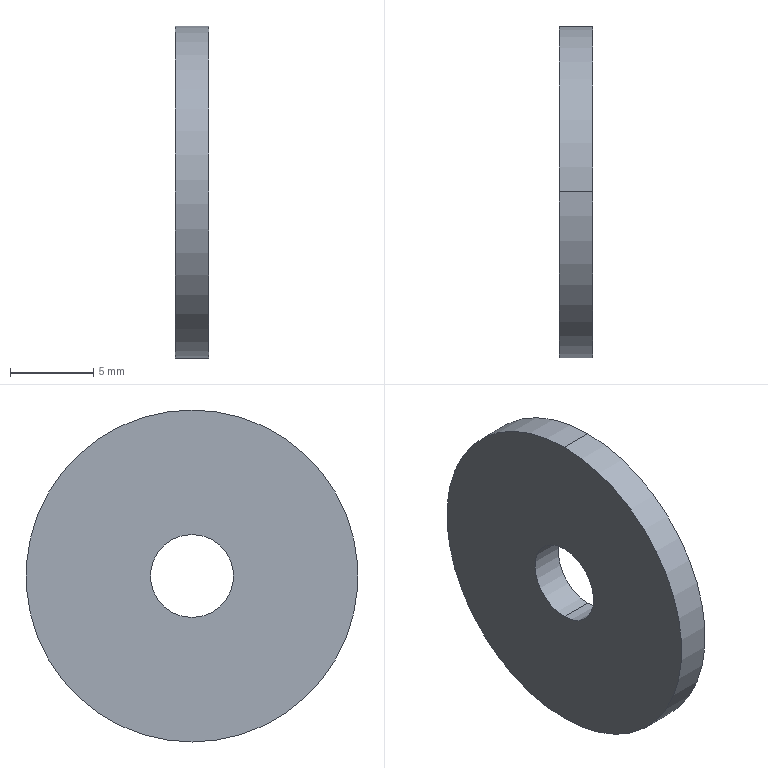Component | SolidWorks | Baffle2-1 | 1 solid | 6 faces | box 2 x 20 x 20 mm | volume 589 mm3 | cylinder 4 | plane 2 | commonest cylinder face diameters 5 x2 20 x2
STEP:
#1=COLOUR_RGB('',0.7922,0.8196,0.9333);
#2=FILL_AREA_STYLE_COLOUR('',#1);
#3=FILL_AREA_STYLE('',(#2));
#4=SURFACE_STYLE_FILL_AREA(#3);
#5=SURFACE_SIDE_STYLE('',(#4));
#6=SURFACE_STYLE_USAGE(.BOTH.,#5);
#7=PRESENTATION_STYLE_ASSIGNMENT((#6));
#8=CARTESIAN_POINT('',(-9.665,5.032,3.217));
#9=VERTEX_POINT('',#8);
#10=CARTESIAN_POINT('',(-9.665,5.032,3.02));
#11=VERTEX_POINT('',#10);
#12=CARTESIAN_POINT('',(-9.665,5.032,3.119));
#13=DIRECTION('',(1.,0.,0.));
#14=DIRECTION('',(0.,0.,-1.));
#15=AXIS2_PLACEMENT_3D('',#12,#13,#14);
#16=CIRCLE('',#15,0.09843);
#17=EDGE_CURVE('',#9,#11,#16,.T.);
#18=ORIENTED_EDGE('',*,*,#17,.F.);
#19=CARTESIAN_POINT('',(-9.587,5.032,3.217));
#20=VERTEX_POINT('',#19);
#21=CARTESIAN_POINT('',(-9.665,5.032,3.217));
#22=DIRECTION('',(1.,0.,0.));
#23=VECTOR('',#22,39.37);
#24=LINE('',#21,#23);
#25=EDGE_CURVE('',#9,#20,#24,.T.);
#26=ORIENTED_EDGE('',*,*,#25,.T.);
#27=CARTESIAN_POINT('',(-9.587,5.032,3.02));
#28=VERTEX_POINT('',#27);
#29=CARTESIAN_POINT('',(-9.587,5.032,3.119));
#30=DIRECTION('',(1.,0.,0.));
#31=DIRECTION('',(0.,0.,-1.));
#32=AXIS2_PLACEMENT_3D('',#29,#30,#31);
#33=CIRCLE('',#32,0.09843);
#34=EDGE_CURVE('',#20,#28,#33,.T.);
#35=ORIENTED_EDGE('',*,*,#34,.T.);
#36=CARTESIAN_POINT('',(-9.665,5.032,3.02));
#37=DIRECTION('',(1.,0.,0.));
#38=VECTOR('',#37,39.37);
#39=LINE('',#36,#38);
#40=EDGE_CURVE('',#11,#28,#39,.T.);
#41=ORIENTED_EDGE('',*,*,#40,.F.);
#42=EDGE_LOOP('',(#18,#26,#35,#41));
#43=FACE_OUTER_BOUND('',#42,.T.);
#44=CARTESIAN_POINT('',(-9.665,5.032,3.119));
#45=DIRECTION('',(1.,0.,0.));
#46=DIRECTION('',(0.,0.,-1.));
#47=AXIS2_PLACEMENT_3D('',#44,#45,#46);
#48=CYLINDRICAL_SURFACE('',#47,0.09843);
#49=ADVANCED_FACE('',(#43),#48,.F.);
#50=CARTESIAN_POINT('',(-9.665,5.032,2.725));
#51=VERTEX_POINT('',#50);
#52=CARTESIAN_POINT('',(-9.665,5.032,3.512));
#53=VERTEX_POINT('',#52);
#54=CARTESIAN_POINT('',(-9.665,5.032,3.119));
#55=DIRECTION('',(1.,0.,0.));
#56=DIRECTION('',(0.,0.,-1.));
#57=AXIS2_PLACEMENT_3D('',#54,#55,#56);
#58=CIRCLE('',#57,0.3937);
#59=EDGE_CURVE('',#51,#53,#58,.T.);
#60=ORIENTED_EDGE('',*,*,#59,.T.);
#61=CARTESIAN_POINT('',(-9.587,5.032,3.512));
#62=VERTEX_POINT('',#61);
#63=CARTESIAN_POINT('',(-9.665,5.032,3.512));
#64=DIRECTION('',(1.,0.,0.));
#65=VECTOR('',#64,39.37);
#66=LINE('',#63,#65);
#67=EDGE_CURVE('',#53,#62,#66,.T.);
#68=ORIENTED_EDGE('',*,*,#67,.T.);
#69=CARTESIAN_POINT('',(-9.587,5.032,2.725));
#70=VERTEX_POINT('',#69);
#71=CARTESIAN_POINT('',(-9.587,5.032,3.119));
#72=DIRECTION('',(1.,0.,0.));
#73=DIRECTION('',(0.,0.,-1.));
#74=AXIS2_PLACEMENT_3D('',#71,#72,#73);
#75=CIRCLE('',#74,0.3937);
#76=EDGE_CURVE('',#70,#62,#75,.T.);
#77=ORIENTED_EDGE('',*,*,#76,.F.);
#78=CARTESIAN_POINT('',(-9.665,5.032,2.725));
#79=DIRECTION('',(1.,0.,0.));
#80=VECTOR('',#79,39.37);
#81=LINE('',#78,#80);
#82=EDGE_CURVE('',#51,#70,#81,.T.);
#83=ORIENTED_EDGE('',*,*,#82,.F.);
#84=EDGE_LOOP('',(#60,#68,#77,#83));
#85=FACE_OUTER_BOUND('',#84,.T.);
#86=CARTESIAN_POINT('',(-9.665,5.032,3.119));
#87=DIRECTION('',(1.,0.,0.));
#88=DIRECTION('',(0.,0.,-1.));
#89=AXIS2_PLACEMENT_3D('',#86,#87,#88);
#90=CYLINDRICAL_SURFACE('',#89,0.3937);
#91=ADVANCED_FACE('',(#85),#90,.T.);
#92=ORIENTED_EDGE('',*,*,#67,.F.);
#93=CARTESIAN_POINT('',(-9.665,5.032,3.119));
#94=DIRECTION('',(1.,0.,0.));
#95=DIRECTION('',(0.,0.,-1.));
#96=AXIS2_PLACEMENT_3D('',#93,#94,#95);
#97=CIRCLE('',#96,0.3937);
#98=EDGE_CURVE('',#53,#51,#97,.T.);
#99=ORIENTED_EDGE('',*,*,#98,.T.);
#100=ORIENTED_EDGE('',*,*,#82,.T.);
#101=CARTESIAN_POINT('',(-9.587,5.032,3.119));
#102=DIRECTION('',(1.,0.,0.));
#103=DIRECTION('',(0.,0.,-1.));
#104=AXIS2_PLACEMENT_3D('',#101,#102,#103);
#105=CIRCLE('',#104,0.3937);
#106=EDGE_CURVE('',#62,#70,#105,.T.);
#107=ORIENTED_EDGE('',*,*,#106,.F.);
#108=EDGE_LOOP('',(#92,#99,#100,#107));
#109=FACE_OUTER_BOUND('',#108,.T.);
#110=CARTESIAN_POINT('',(-9.665,5.032,3.119));
#111=DIRECTION('',(1.,0.,0.));
#112=DIRECTION('',(0.,0.,-1.));
#113=AXIS2_PLACEMENT_3D('',#110,#111,#112);
#114=CYLINDRICAL_SURFACE('',#113,0.3937);
#115=ADVANCED_FACE('',(#109),#114,.T.);
#116=CARTESIAN_POINT('',(-9.665,5.032,3.119));
#117=DIRECTION('',(1.,0.,0.));
#118=DIRECTION('',(0.,0.,-1.));
#119=AXIS2_PLACEMENT_3D('',#116,#117,#118);
#120=CIRCLE('',#119,0.09843);
#121=EDGE_CURVE('',#11,#9,#120,.T.);
#122=ORIENTED_EDGE('',*,*,#121,.T.);
#123=ORIENTED_EDGE('',*,*,#17,.T.);
#124=EDGE_LOOP('',(#122,#123));
#125=FACE_BOUND('',#124,.T.);
#126=ORIENTED_EDGE('',*,*,#59,.F.);
#127=ORIENTED_EDGE('',*,*,#98,.F.);
#128=EDGE_LOOP('',(#126,#127));
#129=FACE_OUTER_BOUND('',#128,.T.);
#130=CARTESIAN_POINT('',(-9.665,5.032,3.119));
#131=DIRECTION('',(1.,0.,0.));
#132=DIRECTION('',(0.,0.,-1.));
#133=AXIS2_PLACEMENT_3D('',#130,#131,#132);
#134=PLANE('',#133);
#135=ADVANCED_FACE('',(#125,#129),#134,.F.);
#136=CARTESIAN_POINT('',(-9.587,5.032,3.119));
#137=DIRECTION('',(1.,0.,0.));
#138=DIRECTION('',(0.,0.,-1.));
#139=AXIS2_PLACEMENT_3D('',#136,#137,#138);
#140=CIRCLE('',#139,0.09843);
#141=EDGE_CURVE('',#28,#20,#140,.T.);
#142=ORIENTED_EDGE('',*,*,#141,.F.);
#143=ORIENTED_EDGE('',*,*,#34,.F.);
#144=EDGE_LOOP('',(#142,#143));
#145=FACE_BOUND('',#144,.T.);
#146=ORIENTED_EDGE('',*,*,#76,.T.);
#147=ORIENTED_EDGE('',*,*,#106,.T.);
#148=EDGE_LOOP('',(#146,#147));
#149=FACE_OUTER_BOUND('',#148,.T.);
#150=CARTESIAN_POINT('',(-9.587,5.032,3.119));
#151=DIRECTION('',(1.,0.,0.));
#152=DIRECTION('',(0.,0.,-1.));
#153=AXIS2_PLACEMENT_3D('',#150,#151,#152);
#154=PLANE('',#153);
#155=ADVANCED_FACE('',(#145,#149),#154,.T.);
#156=ORIENTED_EDGE('',*,*,#25,.F.);
#157=ORIENTED_EDGE('',*,*,#121,.F.);
#158=ORIENTED_EDGE('',*,*,#40,.T.);
#159=ORIENTED_EDGE('',*,*,#141,.T.);
#160=EDGE_LOOP('',(#156,#157,#158,#159));
#161=FACE_OUTER_BOUND('',#160,.T.);
#162=CARTESIAN_POINT('',(-9.665,5.032,3.119));
#163=DIRECTION('',(1.,0.,0.));
#164=DIRECTION('',(0.,0.,-1.));
#165=AXIS2_PLACEMENT_3D('',#162,#163,#164);
#166=CYLINDRICAL_SURFACE('',#165,0.09843);
#167=ADVANCED_FACE('',(#161),#166,.F.);
#168=CLOSED_SHELL('',(#49,#91,#115,#135,#155,#167));
#169=MANIFOLD_SOLID_BREP('',#168);
#170=STYLED_ITEM('',(#7),#169);
#171=(LENGTH_UNIT()NAMED_UNIT(*)SI_UNIT($,.METRE.));
#172=LENGTH_MEASURE_WITH_UNIT(LENGTH_MEASURE(0.0254),#171);
#173=DIMENSIONAL_EXPONENTS(1.,0.,0.,0.,0.,0.,0.);
#174=(CONVERSION_BASED_UNIT('',#172)LENGTH_UNIT()NAMED_UNIT(#173));
#175=UNCERTAINTY_MEASURE_WITH_UNIT(LENGTH_MEASURE(0.00001),#174,'','');
#176=(NAMED_UNIT(*)PLANE_ANGLE_UNIT()SI_UNIT($,.RADIAN.));
#177=(NAMED_UNIT(*)SI_UNIT($,.STERADIAN.)SOLID_ANGLE_UNIT());
#178=(GEOMETRIC_REPRESENTATION_CONTEXT(3)GLOBAL_UNCERTAINTY_ASSIGNED_CONTEXT((#175))GLOBAL_UNIT_ASSIGNED_CONTEXT((#174,#176,#177))REPRESENTATION_CONTEXT('',''));
#179=MECHANICAL_DESIGN_GEOMETRIC_PRESENTATION_REPRESENTATION('',(#170),#178);
#180=CARTESIAN_POINT('',(0.,0.,0.));
#181=DIRECTION('',(0.,0.,1.));
#182=DIRECTION('',(1.,0.,0.));
#183=AXIS2_PLACEMENT_3D('',#180,#181,#182);
#184=(LENGTH_UNIT()NAMED_UNIT(*)SI_UNIT($,.METRE.));
#185=LENGTH_MEASURE_WITH_UNIT(LENGTH_MEASURE(0.0254),#184);
#186=DIMENSIONAL_EXPONENTS(1.,0.,0.,0.,0.,0.,0.);
#187=(CONVERSION_BASED_UNIT('',#185)LENGTH_UNIT()NAMED_UNIT(#186));
#188=UNCERTAINTY_MEASURE_WITH_UNIT(LENGTH_MEASURE(0.00001),#187,'','');
#189=(NAMED_UNIT(*)PLANE_ANGLE_UNIT()SI_UNIT($,.RADIAN.));
#190=(NAMED_UNIT(*)SI_UNIT($,.STERADIAN.)SOLID_ANGLE_UNIT());
#191=(GEOMETRIC_REPRESENTATION_CONTEXT(3)GLOBAL_UNCERTAINTY_ASSIGNED_CONTEXT((#188))GLOBAL_UNIT_ASSIGNED_CONTEXT((#187,#189,#190))REPRESENTATION_CONTEXT('',''));
#192=ADVANCED_BREP_SHAPE_REPRESENTATION('',(#169,#183),#191);
#193=PRESENTATION_LAYER_ASSIGNMENT('','',(#170));